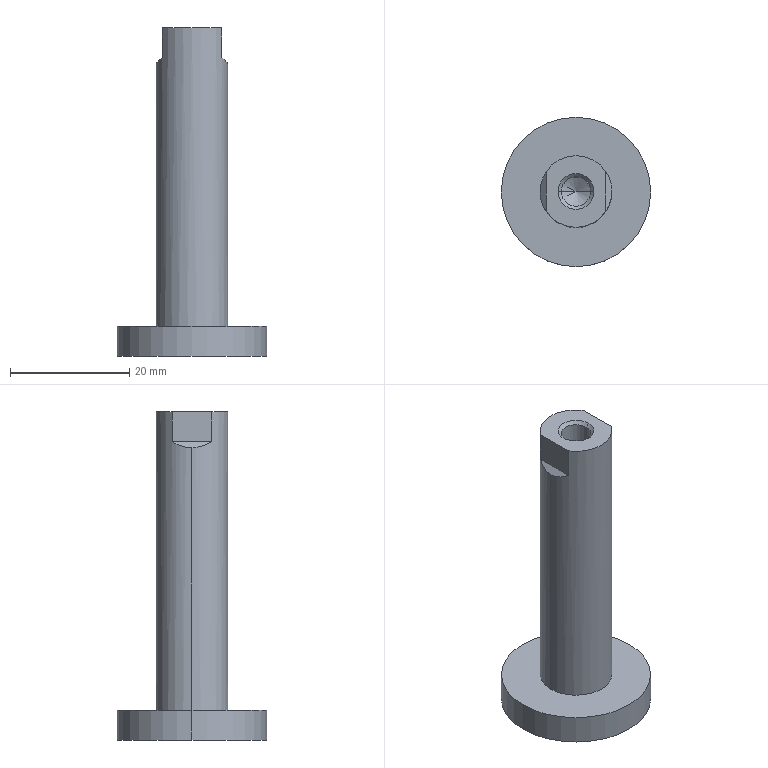Component | SolidWorks | CDQ2B25-35DZ-M9BL-1_CDQ2B25-35M9B(0_0)_CYROD-1 | 1 solid | 17 faces | box 25 x 25 x 55 mm | volume 7821 mm3 | plane 7 | cylinder 6 | cone 4 | commonest cylinder face diameters 25 x2 12 x2 4.917 x2
build123d program:
from build123d import *

# Parameters (mm, degrees)
CUT_EXTRUDE1_DEPTH      = 12
CUT_EXTRUDE1_DEPTH_BACK = 12


with BuildPart() as part:
    # Sketch1 → Revolve1 (revolve)
    with BuildSketch(Plane.XY, mode=Mode.PRIVATE) as revolve1_sk:
        Polygon((8.419, 0), (7, 2.458), (-4.458, 2.458), (-5, 3), (-5, 6), (45, 6), (45, 12.5), (50, 12.5), (50, 0), align=None)
    revolve(revolve1_sk.sketch.rotate(Axis((50, 0, 0), (-1, 0, 0)), 270), axis=Axis((50, 0, 0), (-1, 0, 0)))

    # Sketch2 → Cut-Extrude1 (cut, two sides: drawn at the far end of the back side and taken through both)
    with BuildSketch(Plane(origin=(0, 0, 0), x_dir=(1, 0, 0), z_dir=(0, 1, 0)).offset(-CUT_EXTRUDE1_DEPTH_BACK)):
        Polygon((-10, 10), (-10, -10), (5, -10), (0, -5), (-5, -5), (-5, 5), (0, 5), (5, 10), align=None)
    extrude(amount=CUT_EXTRUDE1_DEPTH + CUT_EXTRUDE1_DEPTH_BACK, mode=Mode.SUBTRACT)


solid = part.part

# Placed as in the assembly
solid = solid.moved(Location((511.649, 139.351, -276.586), (0, 90, 0)))
STEP:
#1=COLOUR_RGB('',0.7922,0.8196,0.9333);
#2=FILL_AREA_STYLE_COLOUR('',#1);
#3=FILL_AREA_STYLE('',(#2));
#4=SURFACE_STYLE_FILL_AREA(#3);
#5=SURFACE_SIDE_STYLE('',(#4));
#6=SURFACE_STYLE_USAGE(.BOTH.,#5);
#7=PRESENTATION_STYLE_ASSIGNMENT((#6));
#8=CARTESIAN_POINT('',(20.636,5.486,-12.858));
#9=VERTEX_POINT('',#8);
#10=CARTESIAN_POINT('',(19.652,5.486,-12.858));
#11=VERTEX_POINT('',#10);
#12=CARTESIAN_POINT('',(20.144,5.486,-12.858));
#13=DIRECTION('',(-0.,-0.,1.));
#14=DIRECTION('',(1.,0.,0.));
#15=AXIS2_PLACEMENT_3D('',#12,#13,#14);
#16=CIRCLE('',#15,0.4921);
#17=EDGE_CURVE('',#9,#11,#16,.T.);
#18=ORIENTED_EDGE('',*,*,#17,.T.);
#19=CARTESIAN_POINT('',(19.652,5.486,-12.661));
#20=VERTEX_POINT('',#19);
#21=CARTESIAN_POINT('',(19.652,5.486,-12.858));
#22=DIRECTION('',(-0.,-0.,1.));
#23=VECTOR('',#22,39.37);
#24=LINE('',#21,#23);
#25=EDGE_CURVE('',#11,#20,#24,.T.);
#26=ORIENTED_EDGE('',*,*,#25,.T.);
#27=CARTESIAN_POINT('',(20.636,5.486,-12.661));
#28=VERTEX_POINT('',#27);
#29=CARTESIAN_POINT('',(20.144,5.486,-12.661));
#30=DIRECTION('',(-0.,-0.,1.));
#31=DIRECTION('',(1.,0.,0.));
#32=AXIS2_PLACEMENT_3D('',#29,#30,#31);
#33=CIRCLE('',#32,0.4921);
#34=EDGE_CURVE('',#28,#20,#33,.T.);
#35=ORIENTED_EDGE('',*,*,#34,.F.);
#36=CARTESIAN_POINT('',(20.636,5.486,-12.858));
#37=DIRECTION('',(-0.,-0.,1.));
#38=VECTOR('',#37,39.37);
#39=LINE('',#36,#38);
#40=EDGE_CURVE('',#9,#28,#39,.T.);
#41=ORIENTED_EDGE('',*,*,#40,.F.);
#42=EDGE_LOOP('',(#18,#26,#35,#41));
#43=FACE_OUTER_BOUND('',#42,.T.);
#44=CARTESIAN_POINT('',(20.144,5.486,-12.858));
#45=DIRECTION('',(-0.,-0.,1.));
#46=DIRECTION('',(1.,0.,0.));
#47=AXIS2_PLACEMENT_3D('',#44,#45,#46);
#48=CYLINDRICAL_SURFACE('',#47,0.4921);
#49=ADVANCED_FACE('',(#43),#48,.T.);
#50=CARTESIAN_POINT('',(20.38,5.486,-12.661));
#51=VERTEX_POINT('',#50);
#52=CARTESIAN_POINT('',(19.907,5.486,-12.661));
#53=VERTEX_POINT('',#52);
#54=CARTESIAN_POINT('',(20.144,5.486,-12.661));
#55=DIRECTION('',(-0.,-0.,1.));
#56=DIRECTION('',(1.,0.,0.));
#57=AXIS2_PLACEMENT_3D('',#54,#55,#56);
#58=CIRCLE('',#57,0.2362);
#59=EDGE_CURVE('',#51,#53,#58,.T.);
#60=ORIENTED_EDGE('',*,*,#59,.T.);
#61=CARTESIAN_POINT('',(19.907,5.486,-10.929));
#62=VERTEX_POINT('',#61);
#63=CARTESIAN_POINT('',(19.907,5.486,-12.858));
#64=DIRECTION('',(-0.,-0.,1.));
#65=VECTOR('',#64,39.37);
#66=LINE('',#63,#65);
#67=EDGE_CURVE('',#53,#62,#66,.T.);
#68=ORIENTED_EDGE('',*,*,#67,.T.);
#69=CARTESIAN_POINT('',(19.947,5.617,-10.889));
#70=VERTEX_POINT('',#69);
#71=CARTESIAN_POINT('',(19.907,5.486,-10.929));
#72=CARTESIAN_POINT('',(19.907,5.533,-10.929));
#73=CARTESIAN_POINT('',(19.921,5.578,-10.915));
#74=CARTESIAN_POINT('',(19.947,5.617,-10.889));
#75=(BOUNDED_CURVE()B_SPLINE_CURVE(3,(#71,#72,#73,#74),.UNSPECIFIED.,.F.,.T.)B_SPLINE_CURVE_WITH_KNOTS((4,4),(3.142,3.727),.UNSPECIFIED.)CURVE()GEOMETRIC_REPRESENTATION_ITEM()RATIONAL_B_SPLINE_CURVE((1.,0.9716,0.9716,1.))REPRESENTATION_ITEM(''));
#76=EDGE_CURVE('',#62,#70,#75,.T.);
#77=ORIENTED_EDGE('',*,*,#76,.T.);
#78=CARTESIAN_POINT('',(19.947,5.617,-10.692));
#79=VERTEX_POINT('',#78);
#80=CARTESIAN_POINT('',(19.947,5.617,-12.858));
#81=DIRECTION('',(-0.,-0.,1.));
#82=VECTOR('',#81,39.37);
#83=LINE('',#80,#82);
#84=EDGE_CURVE('',#70,#79,#83,.T.);
#85=ORIENTED_EDGE('',*,*,#84,.T.);
#86=CARTESIAN_POINT('',(20.341,5.617,-10.692));
#87=VERTEX_POINT('',#86);
#88=CARTESIAN_POINT('',(20.144,5.486,-10.692));
#89=DIRECTION('',(-0.,-0.,1.));
#90=DIRECTION('',(1.,0.,0.));
#91=AXIS2_PLACEMENT_3D('',#88,#89,#90);
#92=CIRCLE('',#91,0.2362);
#93=EDGE_CURVE('',#87,#79,#92,.T.);
#94=ORIENTED_EDGE('',*,*,#93,.F.);
#95=CARTESIAN_POINT('',(20.341,5.617,-10.889));
#96=VERTEX_POINT('',#95);
#97=CARTESIAN_POINT('',(20.341,5.617,-12.858));
#98=DIRECTION('',(0.,0.,-1.));
#99=VECTOR('',#98,39.37);
#100=LINE('',#97,#99);
#101=EDGE_CURVE('',#87,#96,#100,.T.);
#102=ORIENTED_EDGE('',*,*,#101,.T.);
#103=CARTESIAN_POINT('',(20.38,5.486,-10.929));
#104=VERTEX_POINT('',#103);
#105=CARTESIAN_POINT('',(20.341,5.617,-10.889));
#106=CARTESIAN_POINT('',(20.366,5.578,-10.915));
#107=CARTESIAN_POINT('',(20.38,5.533,-10.929));
#108=CARTESIAN_POINT('',(20.38,5.486,-10.929));
#109=(BOUNDED_CURVE()B_SPLINE_CURVE(3,(#105,#106,#107,#108),.UNSPECIFIED.,.F.,.T.)B_SPLINE_CURVE_WITH_KNOTS((4,4),(2.556,3.142),.UNSPECIFIED.)CURVE()GEOMETRIC_REPRESENTATION_ITEM()RATIONAL_B_SPLINE_CURVE((1.,0.9716,0.9716,1.))REPRESENTATION_ITEM(''));
#110=EDGE_CURVE('',#96,#104,#109,.T.);
#111=ORIENTED_EDGE('',*,*,#110,.T.);
#112=CARTESIAN_POINT('',(20.38,5.486,-12.858));
#113=DIRECTION('',(-0.,-0.,1.));
#114=VECTOR('',#113,39.37);
#115=LINE('',#112,#114);
#116=EDGE_CURVE('',#51,#104,#115,.T.);
#117=ORIENTED_EDGE('',*,*,#116,.F.);
#118=EDGE_LOOP('',(#60,#68,#77,#85,#94,#102,#111,#117));
#119=FACE_OUTER_BOUND('',#118,.T.);
#120=CARTESIAN_POINT('',(20.144,5.486,-12.858));
#121=DIRECTION('',(-0.,-0.,1.));
#122=DIRECTION('',(1.,0.,0.));
#123=AXIS2_PLACEMENT_3D('',#120,#121,#122);
#124=CYLINDRICAL_SURFACE('',#123,0.2362);
#125=ADVANCED_FACE('',(#119),#124,.T.);
#126=CARTESIAN_POINT('',(20.047,5.486,-10.714));
#127=VERTEX_POINT('',#126);
#128=CARTESIAN_POINT('',(20.24,5.486,-10.714));
#129=VERTEX_POINT('',#128);
#130=CARTESIAN_POINT('',(20.144,5.486,-10.714));
#131=DIRECTION('',(-0.,-0.,1.));
#132=DIRECTION('',(1.,0.,0.));
#133=AXIS2_PLACEMENT_3D('',#130,#131,#132);
#134=CIRCLE('',#133,0.09679);
#135=EDGE_CURVE('',#127,#129,#134,.T.);
#136=ORIENTED_EDGE('',*,*,#135,.F.);
#137=CARTESIAN_POINT('',(20.026,5.486,-10.692));
#138=VERTEX_POINT('',#137);
#139=CARTESIAN_POINT('',(20.026,5.486,-10.692));
#140=DIRECTION('',(-0.7071,0.,0.7071));
#141=VECTOR('',#140,39.37);
#142=LINE('',#139,#141);
#143=EDGE_CURVE('',#127,#138,#142,.T.);
#144=ORIENTED_EDGE('',*,*,#143,.T.);
#145=CARTESIAN_POINT('',(20.262,5.486,-10.692));
#146=VERTEX_POINT('',#145);
#147=CARTESIAN_POINT('',(20.144,5.486,-10.692));
#148=DIRECTION('',(-0.,-0.,1.));
#149=DIRECTION('',(1.,0.,0.));
#150=AXIS2_PLACEMENT_3D('',#147,#148,#149);
#151=CIRCLE('',#150,0.1181);
#152=EDGE_CURVE('',#138,#146,#151,.T.);
#153=ORIENTED_EDGE('',*,*,#152,.T.);
#154=CARTESIAN_POINT('',(20.262,5.486,-10.692));
#155=DIRECTION('',(0.7071,-0.,0.7071));
#156=VECTOR('',#155,39.37);
#157=LINE('',#154,#156);
#158=EDGE_CURVE('',#129,#146,#157,.T.);
#159=ORIENTED_EDGE('',*,*,#158,.F.);
#160=EDGE_LOOP('',(#136,#144,#153,#159));
#161=FACE_OUTER_BOUND('',#160,.T.);
#162=CARTESIAN_POINT('',(20.144,5.486,-10.692));
#163=DIRECTION('',(-0.,-0.,1.));
#164=DIRECTION('',(1.,0.,0.));
#165=AXIS2_PLACEMENT_3D('',#162,#163,#164);
#166=CONICAL_SURFACE('',#165,0.1181,0.7854);
#167=ADVANCED_FACE('',(#161),#166,.F.);
#168=CARTESIAN_POINT('',(20.047,5.486,-11.165));
#169=VERTEX_POINT('',#168);
#170=CARTESIAN_POINT('',(20.24,5.486,-11.165));
#171=VERTEX_POINT('',#170);
#172=CARTESIAN_POINT('',(20.144,5.486,-11.165));
#173=DIRECTION('',(-0.,-0.,1.));
#174=DIRECTION('',(1.,0.,0.));
#175=AXIS2_PLACEMENT_3D('',#172,#173,#174);
#176=CIRCLE('',#175,0.09679);
#177=EDGE_CURVE('',#169,#171,#176,.T.);
#178=ORIENTED_EDGE('',*,*,#177,.F.);
#179=CARTESIAN_POINT('',(20.047,5.486,-12.858));
#180=DIRECTION('',(-0.,-0.,1.));
#181=VECTOR('',#180,39.37);
#182=LINE('',#179,#181);
#183=EDGE_CURVE('',#169,#127,#182,.T.);
#184=ORIENTED_EDGE('',*,*,#183,.T.);
#185=ORIENTED_EDGE('',*,*,#135,.T.);
#186=CARTESIAN_POINT('',(20.24,5.486,-12.858));
#187=DIRECTION('',(-0.,-0.,1.));
#188=VECTOR('',#187,39.37);
#189=LINE('',#186,#188);
#190=EDGE_CURVE('',#171,#129,#189,.T.);
#191=ORIENTED_EDGE('',*,*,#190,.F.);
#192=EDGE_LOOP('',(#178,#184,#185,#191));
#193=FACE_OUTER_BOUND('',#192,.T.);
#194=CARTESIAN_POINT('',(20.144,5.486,-12.858));
#195=DIRECTION('',(-0.,-0.,1.));
#196=DIRECTION('',(1.,0.,0.));
#197=AXIS2_PLACEMENT_3D('',#194,#195,#196);
#198=CYLINDRICAL_SURFACE('',#197,0.09679);
#199=ADVANCED_FACE('',(#193),#198,.F.);
#200=CARTESIAN_POINT('',(20.144,5.486,-11.221));
#201=VERTEX_POINT('',#200);
#202=CARTESIAN_POINT('',(20.24,5.486,-11.165));
#203=DIRECTION('',(0.866,-0.,0.5));
#204=VECTOR('',#203,39.37);
#205=LINE('',#202,#204);
#206=EDGE_CURVE('',#201,#171,#205,.T.);
#207=ORIENTED_EDGE('',*,*,#206,.F.);
#208=CARTESIAN_POINT('',(20.047,5.486,-11.165));
#209=DIRECTION('',(-0.866,0.,0.5));
#210=VECTOR('',#209,39.37);
#211=LINE('',#208,#210);
#212=EDGE_CURVE('',#201,#169,#211,.T.);
#213=ORIENTED_EDGE('',*,*,#212,.T.);
#214=ORIENTED_EDGE('',*,*,#177,.T.);
#215=EDGE_LOOP('',(#207,#213,#214));
#216=FACE_OUTER_BOUND('',#215,.T.);
#217=CARTESIAN_POINT('',(20.144,5.486,-11.165));
#218=DIRECTION('',(-0.,-0.,1.));
#219=DIRECTION('',(1.,0.,0.));
#220=AXIS2_PLACEMENT_3D('',#217,#218,#219);
#221=CONICAL_SURFACE('',#220,0.09679,1.047);
#222=ADVANCED_FACE('',(#216),#221,.F.);
#223=ORIENTED_EDGE('',*,*,#212,.F.);
#224=ORIENTED_EDGE('',*,*,#206,.T.);
#225=CARTESIAN_POINT('',(20.144,5.486,-11.165));
#226=DIRECTION('',(-0.,-0.,1.));
#227=DIRECTION('',(1.,0.,0.));
#228=AXIS2_PLACEMENT_3D('',#225,#226,#227);
#229=CIRCLE('',#228,0.09679);
#230=EDGE_CURVE('',#171,#169,#229,.T.);
#231=ORIENTED_EDGE('',*,*,#230,.T.);
#232=EDGE_LOOP('',(#223,#224,#231));
#233=FACE_OUTER_BOUND('',#232,.T.);
#234=CARTESIAN_POINT('',(20.144,5.486,-11.165));
#235=DIRECTION('',(-0.,-0.,1.));
#236=DIRECTION('',(1.,0.,0.));
#237=AXIS2_PLACEMENT_3D('',#234,#235,#236);
#238=CONICAL_SURFACE('',#237,0.09679,1.047);
#239=ADVANCED_FACE('',(#233),#238,.F.);
#240=ORIENTED_EDGE('',*,*,#183,.F.);
#241=ORIENTED_EDGE('',*,*,#230,.F.);
#242=ORIENTED_EDGE('',*,*,#190,.T.);
#243=CARTESIAN_POINT('',(20.144,5.486,-10.714));
#244=DIRECTION('',(-0.,-0.,1.));
#245=DIRECTION('',(1.,0.,0.));
#246=AXIS2_PLACEMENT_3D('',#243,#244,#245);
#247=CIRCLE('',#246,0.09679);
#248=EDGE_CURVE('',#129,#127,#247,.T.);
#249=ORIENTED_EDGE('',*,*,#248,.T.);
#250=EDGE_LOOP('',(#240,#241,#242,#249));
#251=FACE_OUTER_BOUND('',#250,.T.);
#252=CARTESIAN_POINT('',(20.144,5.486,-12.858));
#253=DIRECTION('',(-0.,-0.,1.));
#254=DIRECTION('',(1.,0.,0.));
#255=AXIS2_PLACEMENT_3D('',#252,#253,#254);
#256=CYLINDRICAL_SURFACE('',#255,0.09679);
#257=ADVANCED_FACE('',(#251),#256,.F.);
#258=ORIENTED_EDGE('',*,*,#143,.F.);
#259=ORIENTED_EDGE('',*,*,#248,.F.);
#260=ORIENTED_EDGE('',*,*,#158,.T.);
#261=CARTESIAN_POINT('',(20.144,5.486,-10.692));
#262=DIRECTION('',(-0.,-0.,1.));
#263=DIRECTION('',(1.,0.,0.));
#264=AXIS2_PLACEMENT_3D('',#261,#262,#263);
#265=CIRCLE('',#264,0.1181);
#266=EDGE_CURVE('',#146,#138,#265,.T.);
#267=ORIENTED_EDGE('',*,*,#266,.T.);
#268=EDGE_LOOP('',(#258,#259,#260,#267));
#269=FACE_OUTER_BOUND('',#268,.T.);
#270=CARTESIAN_POINT('',(20.144,5.486,-10.692));
#271=DIRECTION('',(-0.,-0.,1.));
#272=DIRECTION('',(1.,0.,0.));
#273=AXIS2_PLACEMENT_3D('',#270,#271,#272);
#274=CONICAL_SURFACE('',#273,0.1181,0.7854);
#275=ADVANCED_FACE('',(#269),#274,.F.);
#276=ORIENTED_EDGE('',*,*,#266,.F.);
#277=ORIENTED_EDGE('',*,*,#152,.F.);
#278=EDGE_LOOP('',(#276,#277));
#279=FACE_BOUND('',#278,.T.);
#280=ORIENTED_EDGE('',*,*,#93,.T.);
#281=CARTESIAN_POINT('',(19.947,5.356,-10.692));
#282=VERTEX_POINT('',#281);
#283=CARTESIAN_POINT('',(19.947,5.014,-10.692));
#284=DIRECTION('',(-0.,1.,0.));
#285=VECTOR('',#284,39.37);
#286=LINE('',#283,#285);
#287=EDGE_CURVE('',#282,#79,#286,.T.);
#288=ORIENTED_EDGE('',*,*,#287,.F.);
#289=CARTESIAN_POINT('',(20.341,5.356,-10.692));
#290=VERTEX_POINT('',#289);
#291=CARTESIAN_POINT('',(20.144,5.486,-10.692));
#292=DIRECTION('',(-0.,-0.,1.));
#293=DIRECTION('',(1.,0.,0.));
#294=AXIS2_PLACEMENT_3D('',#291,#292,#293);
#295=CIRCLE('',#294,0.2362);
#296=EDGE_CURVE('',#282,#290,#295,.T.);
#297=ORIENTED_EDGE('',*,*,#296,.T.);
#298=CARTESIAN_POINT('',(20.341,5.014,-10.692));
#299=DIRECTION('',(-0.,1.,0.));
#300=VECTOR('',#299,39.37);
#301=LINE('',#298,#300);
#302=EDGE_CURVE('',#290,#87,#301,.T.);
#303=ORIENTED_EDGE('',*,*,#302,.T.);
#304=EDGE_LOOP('',(#280,#288,#297,#303));
#305=FACE_OUTER_BOUND('',#304,.T.);
#306=CARTESIAN_POINT('',(20.144,5.604,-10.692));
#307=DIRECTION('',(0.,0.,-1.));
#308=DIRECTION('',(-1.,0.,-0.));
#309=AXIS2_PLACEMENT_3D('',#306,#307,#308);
#310=PLANE('',#309);
#311=ADVANCED_FACE('',(#279,#305),#310,.F.);
#312=ORIENTED_EDGE('',*,*,#67,.F.);
#313=CARTESIAN_POINT('',(20.144,5.486,-12.661));
#314=DIRECTION('',(-0.,-0.,1.));
#315=DIRECTION('',(1.,0.,0.));
#316=AXIS2_PLACEMENT_3D('',#313,#314,#315);
#317=CIRCLE('',#316,0.2362);
#318=EDGE_CURVE('',#53,#51,#317,.T.);
#319=ORIENTED_EDGE('',*,*,#318,.T.);
#320=ORIENTED_EDGE('',*,*,#116,.T.);
#321=CARTESIAN_POINT('',(20.341,5.356,-10.889));
#322=VERTEX_POINT('',#321);
#323=CARTESIAN_POINT('',(20.38,5.486,-10.929));
#324=CARTESIAN_POINT('',(20.38,5.439,-10.929));
#325=CARTESIAN_POINT('',(20.366,5.395,-10.915));
#326=CARTESIAN_POINT('',(20.341,5.356,-10.889));
#327=(BOUNDED_CURVE()B_SPLINE_CURVE(3,(#323,#324,#325,#326),.UNSPECIFIED.,.F.,.T.)B_SPLINE_CURVE_WITH_KNOTS((4,4),(3.142,3.727),.UNSPECIFIED.)CURVE()GEOMETRIC_REPRESENTATION_ITEM()RATIONAL_B_SPLINE_CURVE((1.,0.9716,0.9716,1.))REPRESENTATION_ITEM(''));
#328=EDGE_CURVE('',#104,#322,#327,.T.);
#329=ORIENTED_EDGE('',*,*,#328,.T.);
#330=CARTESIAN_POINT('',(20.341,5.356,-12.858));
#331=DIRECTION('',(-0.,-0.,1.));
#332=VECTOR('',#331,39.37);
#333=LINE('',#330,#332);
#334=EDGE_CURVE('',#322,#290,#333,.T.);
#335=ORIENTED_EDGE('',*,*,#334,.T.);
#336=ORIENTED_EDGE('',*,*,#296,.F.);
#337=CARTESIAN_POINT('',(19.947,5.356,-10.889));
#338=VERTEX_POINT('',#337);
#339=CARTESIAN_POINT('',(19.947,5.356,-12.858));
#340=DIRECTION('',(0.,0.,-1.));
#341=VECTOR('',#340,39.37);
#342=LINE('',#339,#341);
#343=EDGE_CURVE('',#282,#338,#342,.T.);
#344=ORIENTED_EDGE('',*,*,#343,.T.);
#345=CARTESIAN_POINT('',(19.947,5.356,-10.889));
#346=CARTESIAN_POINT('',(19.921,5.395,-10.915));
#347=CARTESIAN_POINT('',(19.907,5.439,-10.929));
#348=CARTESIAN_POINT('',(19.907,5.486,-10.929));
#349=(BOUNDED_CURVE()B_SPLINE_CURVE(3,(#345,#346,#347,#348),.UNSPECIFIED.,.F.,.T.)B_SPLINE_CURVE_WITH_KNOTS((4,4),(2.556,3.142),.UNSPECIFIED.)CURVE()GEOMETRIC_REPRESENTATION_ITEM()RATIONAL_B_SPLINE_CURVE((1.,0.9716,0.9716,1.))REPRESENTATION_ITEM(''));
#350=EDGE_CURVE('',#338,#62,#349,.T.);
#351=ORIENTED_EDGE('',*,*,#350,.T.);
#352=EDGE_LOOP('',(#312,#319,#320,#329,#335,#336,#344,#351));
#353=FACE_OUTER_BOUND('',#352,.T.);
#354=CARTESIAN_POINT('',(20.144,5.486,-12.858));
#355=DIRECTION('',(-0.,-0.,1.));
#356=DIRECTION('',(1.,0.,0.));
#357=AXIS2_PLACEMENT_3D('',#354,#355,#356);
#358=CYLINDRICAL_SURFACE('',#357,0.2362);
#359=ADVANCED_FACE('',(#353),#358,.T.);
#360=ORIENTED_EDGE('',*,*,#59,.F.);
#361=ORIENTED_EDGE('',*,*,#318,.F.);
#362=EDGE_LOOP('',(#360,#361));
#363=FACE_BOUND('',#362,.T.);
#364=ORIENTED_EDGE('',*,*,#34,.T.);
#365=CARTESIAN_POINT('',(20.144,5.486,-12.661));
#366=DIRECTION('',(-0.,-0.,1.));
#367=DIRECTION('',(1.,0.,0.));
#368=AXIS2_PLACEMENT_3D('',#365,#366,#367);
#369=CIRCLE('',#368,0.4921);
#370=EDGE_CURVE('',#20,#28,#369,.T.);
#371=ORIENTED_EDGE('',*,*,#370,.T.);
#372=EDGE_LOOP('',(#364,#371));
#373=FACE_OUTER_BOUND('',#372,.T.);
#374=CARTESIAN_POINT('',(20.144,5.722,-12.661));
#375=DIRECTION('',(0.,0.,-1.));
#376=DIRECTION('',(-1.,0.,-0.));
#377=AXIS2_PLACEMENT_3D('',#374,#375,#376);
#378=PLANE('',#377);
#379=ADVANCED_FACE('',(#363,#373),#378,.F.);
#380=ORIENTED_EDGE('',*,*,#25,.F.);
#381=CARTESIAN_POINT('',(20.144,5.486,-12.858));
#382=DIRECTION('',(-0.,-0.,1.));
#383=DIRECTION('',(1.,0.,0.));
#384=AXIS2_PLACEMENT_3D('',#381,#382,#383);
#385=CIRCLE('',#384,0.4921);
#386=EDGE_CURVE('',#11,#9,#385,.T.);
#387=ORIENTED_EDGE('',*,*,#386,.T.);
#388=ORIENTED_EDGE('',*,*,#40,.T.);
#389=ORIENTED_EDGE('',*,*,#370,.F.);
#390=EDGE_LOOP('',(#380,#387,#388,#389));
#391=FACE_OUTER_BOUND('',#390,.T.);
#392=CARTESIAN_POINT('',(20.144,5.486,-12.858));
#393=DIRECTION('',(-0.,-0.,1.));
#394=DIRECTION('',(1.,0.,0.));
#395=AXIS2_PLACEMENT_3D('',#392,#393,#394);
#396=CYLINDRICAL_SURFACE('',#395,0.4921);
#397=ADVANCED_FACE('',(#391),#396,.T.);
#398=ORIENTED_EDGE('',*,*,#17,.F.);
#399=ORIENTED_EDGE('',*,*,#386,.F.);
#400=EDGE_LOOP('',(#398,#399));
#401=FACE_OUTER_BOUND('',#400,.T.);
#402=CARTESIAN_POINT('',(20.144,5.978,-12.858));
#403=DIRECTION('',(-0.,-0.,1.));
#404=DIRECTION('',(1.,-0.,0.));
#405=AXIS2_PLACEMENT_3D('',#402,#403,#404);
#406=PLANE('',#405);
#407=ADVANCED_FACE('',(#401),#406,.F.);
#408=CARTESIAN_POINT('',(20.341,5.014,-10.889));
#409=DIRECTION('',(-0.,1.,0.));
#410=VECTOR('',#409,39.37);
#411=LINE('',#408,#410);
#412=EDGE_CURVE('',#322,#96,#411,.T.);
#413=ORIENTED_EDGE('',*,*,#412,.F.);
#414=ORIENTED_EDGE('',*,*,#328,.F.);
#415=ORIENTED_EDGE('',*,*,#110,.F.);
#416=EDGE_LOOP('',(#413,#414,#415));
#417=FACE_OUTER_BOUND('',#416,.T.);
#418=CARTESIAN_POINT('',(20.537,5.014,-11.086));
#419=DIRECTION('',(-0.7071,0.,-0.7071));
#420=DIRECTION('',(-0.7071,-0.,0.7071));
#421=AXIS2_PLACEMENT_3D('',#418,#419,#420);
#422=PLANE('',#421);
#423=ADVANCED_FACE('',(#417),#422,.F.);
#424=ORIENTED_EDGE('',*,*,#412,.T.);
#425=ORIENTED_EDGE('',*,*,#101,.F.);
#426=ORIENTED_EDGE('',*,*,#302,.F.);
#427=ORIENTED_EDGE('',*,*,#334,.F.);
#428=EDGE_LOOP('',(#424,#425,#426,#427));
#429=FACE_OUTER_BOUND('',#428,.T.);
#430=CARTESIAN_POINT('',(20.341,5.014,-10.889));
#431=DIRECTION('',(-1.,0.,-0.));
#432=DIRECTION('',(-0.,-0.,1.));
#433=AXIS2_PLACEMENT_3D('',#430,#431,#432);
#434=PLANE('',#433);
#435=ADVANCED_FACE('',(#429),#434,.F.);
#436=CARTESIAN_POINT('',(19.947,5.014,-10.889));
#437=DIRECTION('',(-0.,1.,0.));
#438=VECTOR('',#437,39.37);
#439=LINE('',#436,#438);
#440=EDGE_CURVE('',#338,#70,#439,.T.);
#441=ORIENTED_EDGE('',*,*,#440,.T.);
#442=ORIENTED_EDGE('',*,*,#76,.F.);
#443=ORIENTED_EDGE('',*,*,#350,.F.);
#444=EDGE_LOOP('',(#441,#442,#443));
#445=FACE_OUTER_BOUND('',#444,.T.);
#446=CARTESIAN_POINT('',(19.947,5.014,-10.889));
#447=DIRECTION('',(0.7071,0.,-0.7071));
#448=DIRECTION('',(-0.7071,0.,-0.7071));
#449=AXIS2_PLACEMENT_3D('',#446,#447,#448);
#450=PLANE('',#449);
#451=ADVANCED_FACE('',(#445),#450,.F.);
#452=ORIENTED_EDGE('',*,*,#440,.F.);
#453=ORIENTED_EDGE('',*,*,#343,.F.);
#454=ORIENTED_EDGE('',*,*,#287,.T.);
#455=ORIENTED_EDGE('',*,*,#84,.F.);
#456=EDGE_LOOP('',(#452,#453,#454,#455));
#457=FACE_OUTER_BOUND('',#456,.T.);
#458=CARTESIAN_POINT('',(19.947,5.014,-10.692));
#459=DIRECTION('',(1.,-0.,0.));
#460=DIRECTION('',(0.,0.,-1.));
#461=AXIS2_PLACEMENT_3D('',#458,#459,#460);
#462=PLANE('',#461);
#463=ADVANCED_FACE('',(#457),#462,.F.);
#464=CLOSED_SHELL('',(#49,#125,#167,#199,#222,#239,#257,#275,#311,#359,#379,#397,#407,#423,#435,#451,#463));
#465=MANIFOLD_SOLID_BREP('',#464);
#466=STYLED_ITEM('',(#7),#465);
#467=PRESENTATION_LAYER_ASSIGNMENT('','',(#466));
#468=CARTESIAN_POINT('',(0.,0.,0.));
#469=DIRECTION('',(0.,0.,1.));
#470=DIRECTION('',(1.,0.,0.));
#471=AXIS2_PLACEMENT_3D('',#468,#469,#470);
#472=(LENGTH_UNIT()NAMED_UNIT(*)SI_UNIT($,.METRE.));
#473=LENGTH_MEASURE_WITH_UNIT(LENGTH_MEASURE(0.0254),#472);
#474=DIMENSIONAL_EXPONENTS(1.,0.,0.,0.,0.,0.,0.);
#475=(CONVERSION_BASED_UNIT('',#473)LENGTH_UNIT()NAMED_UNIT(#474));
#476=UNCERTAINTY_MEASURE_WITH_UNIT(LENGTH_MEASURE(0.00001),#475,'','');
#477=(NAMED_UNIT(*)PLANE_ANGLE_UNIT()SI_UNIT($,.RADIAN.));
#478=(NAMED_UNIT(*)SI_UNIT($,.STERADIAN.)SOLID_ANGLE_UNIT());
#479=(GEOMETRIC_REPRESENTATION_CONTEXT(3)GLOBAL_UNCERTAINTY_ASSIGNED_CONTEXT((#476))GLOBAL_UNIT_ASSIGNED_CONTEXT((#475,#477,#478))REPRESENTATION_CONTEXT('',''));
#480=ADVANCED_BREP_SHAPE_REPRESENTATION('',(#465,#471),#479);
#481=(LENGTH_UNIT()NAMED_UNIT(*)SI_UNIT($,.METRE.));
#482=LENGTH_MEASURE_WITH_UNIT(LENGTH_MEASURE(0.0254),#481);
#483=DIMENSIONAL_EXPONENTS(1.,0.,0.,0.,0.,0.,0.);
#484=(CONVERSION_BASED_UNIT('',#482)LENGTH_UNIT()NAMED_UNIT(#483));
#485=UNCERTAINTY_MEASURE_WITH_UNIT(LENGTH_MEASURE(0.00001),#484,'','');
#486=(NAMED_UNIT(*)PLANE_ANGLE_UNIT()SI_UNIT($,.RADIAN.));
#487=(NAMED_UNIT(*)SI_UNIT($,.STERADIAN.)SOLID_ANGLE_UNIT());
#488=(GEOMETRIC_REPRESENTATION_CONTEXT(3)GLOBAL_UNCERTAINTY_ASSIGNED_CONTEXT((#485))GLOBAL_UNIT_ASSIGNED_CONTEXT((#484,#486,#487))REPRESENTATION_CONTEXT('',''));
#489=MECHANICAL_DESIGN_GEOMETRIC_PRESENTATION_REPRESENTATION('',(#466),#488);